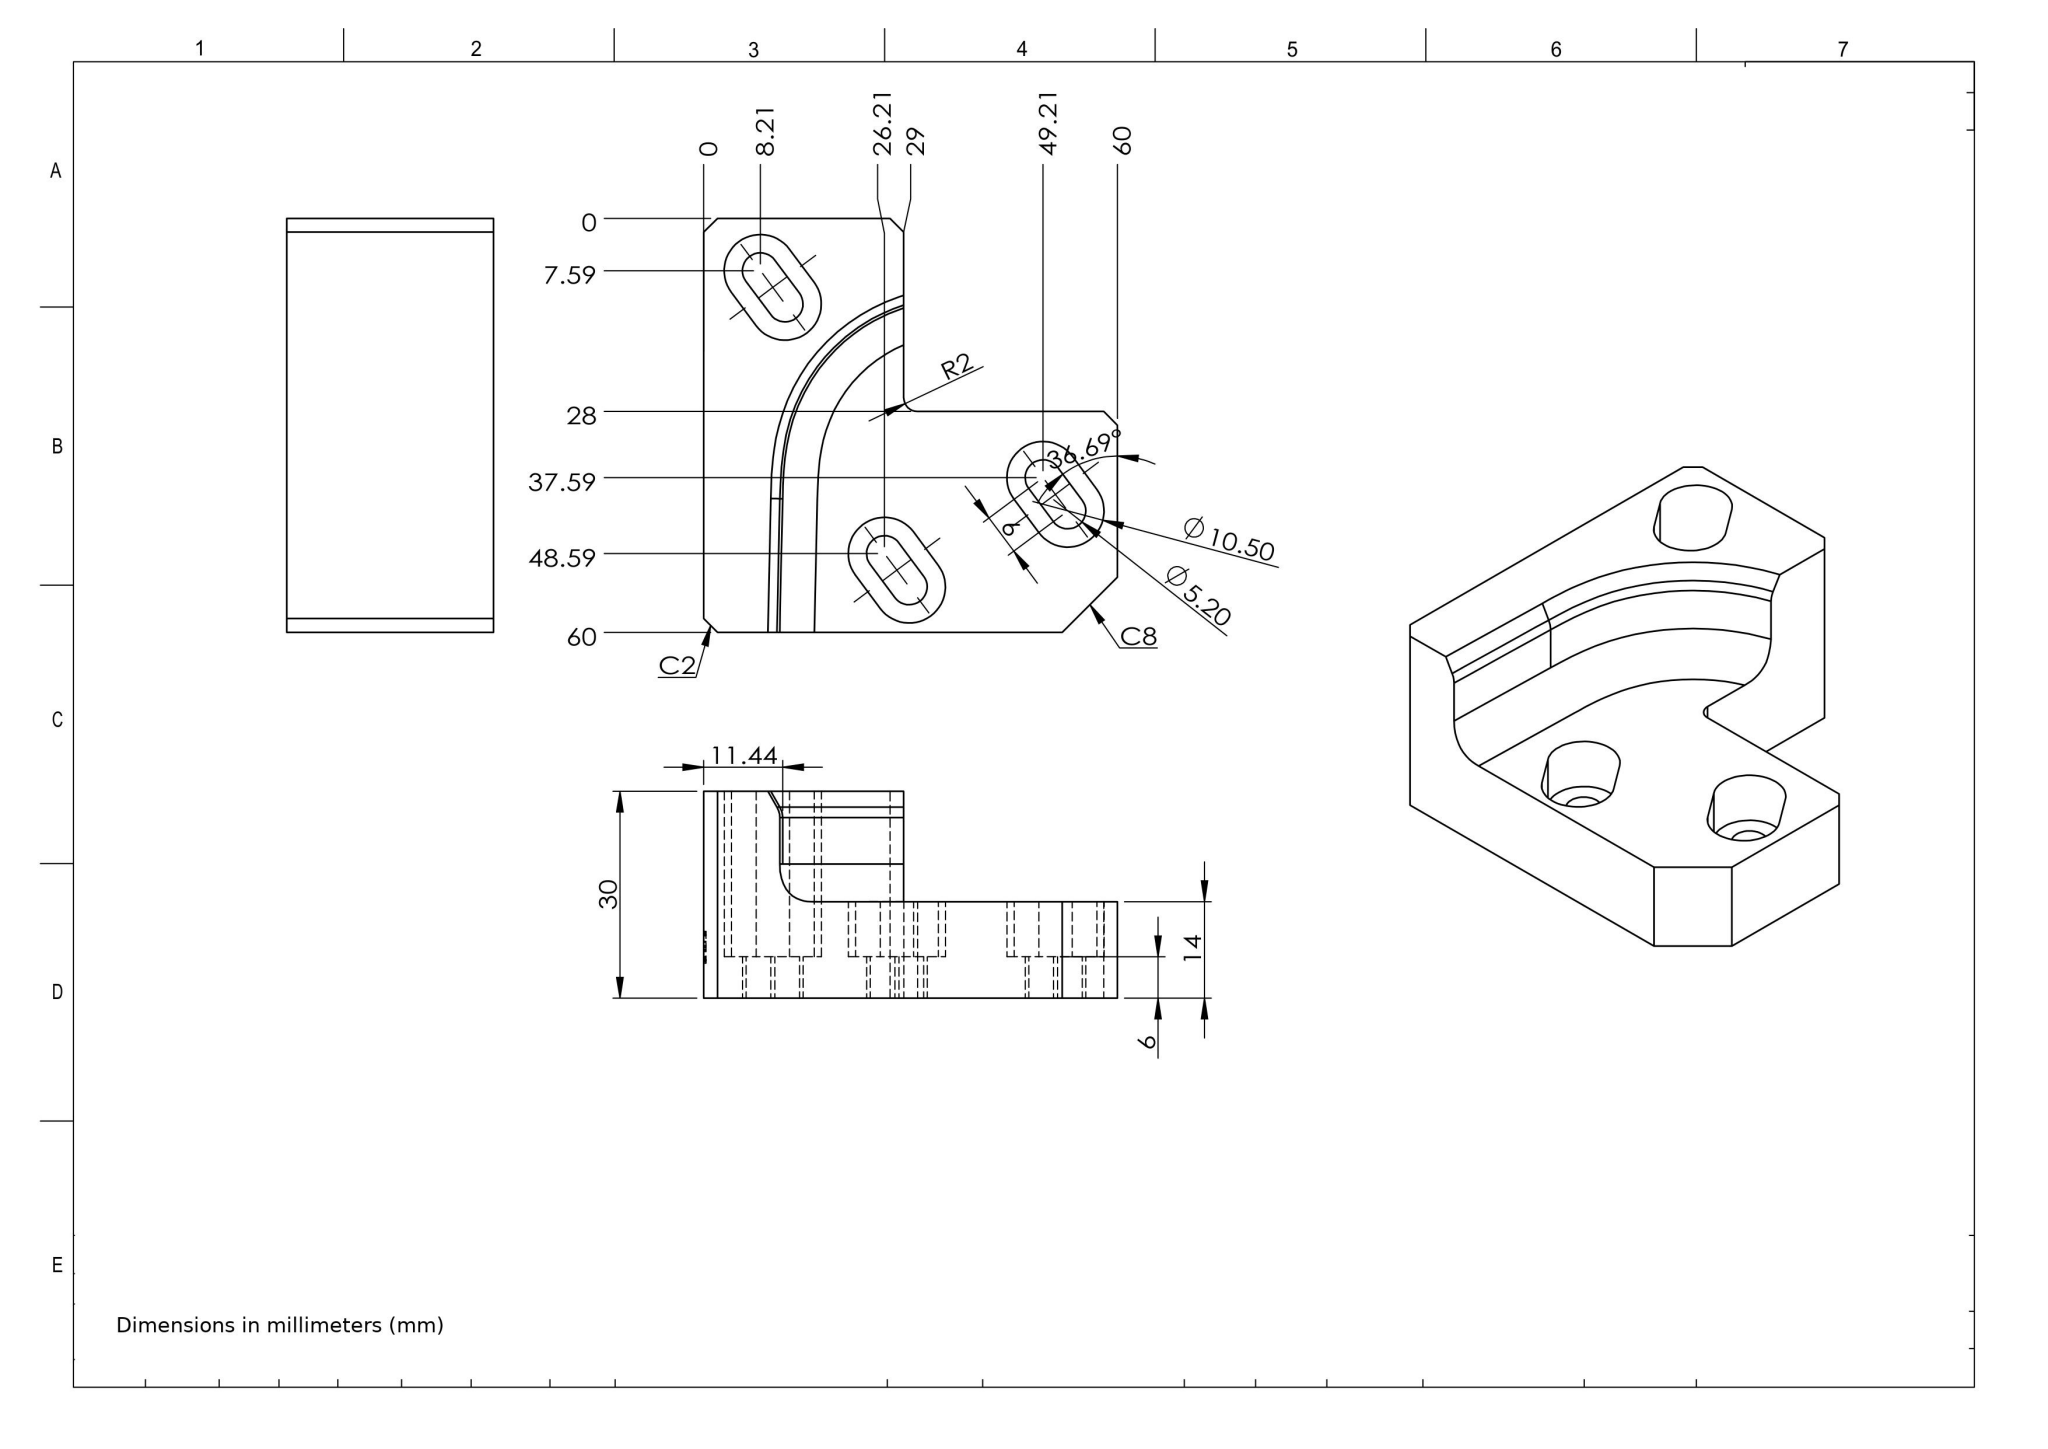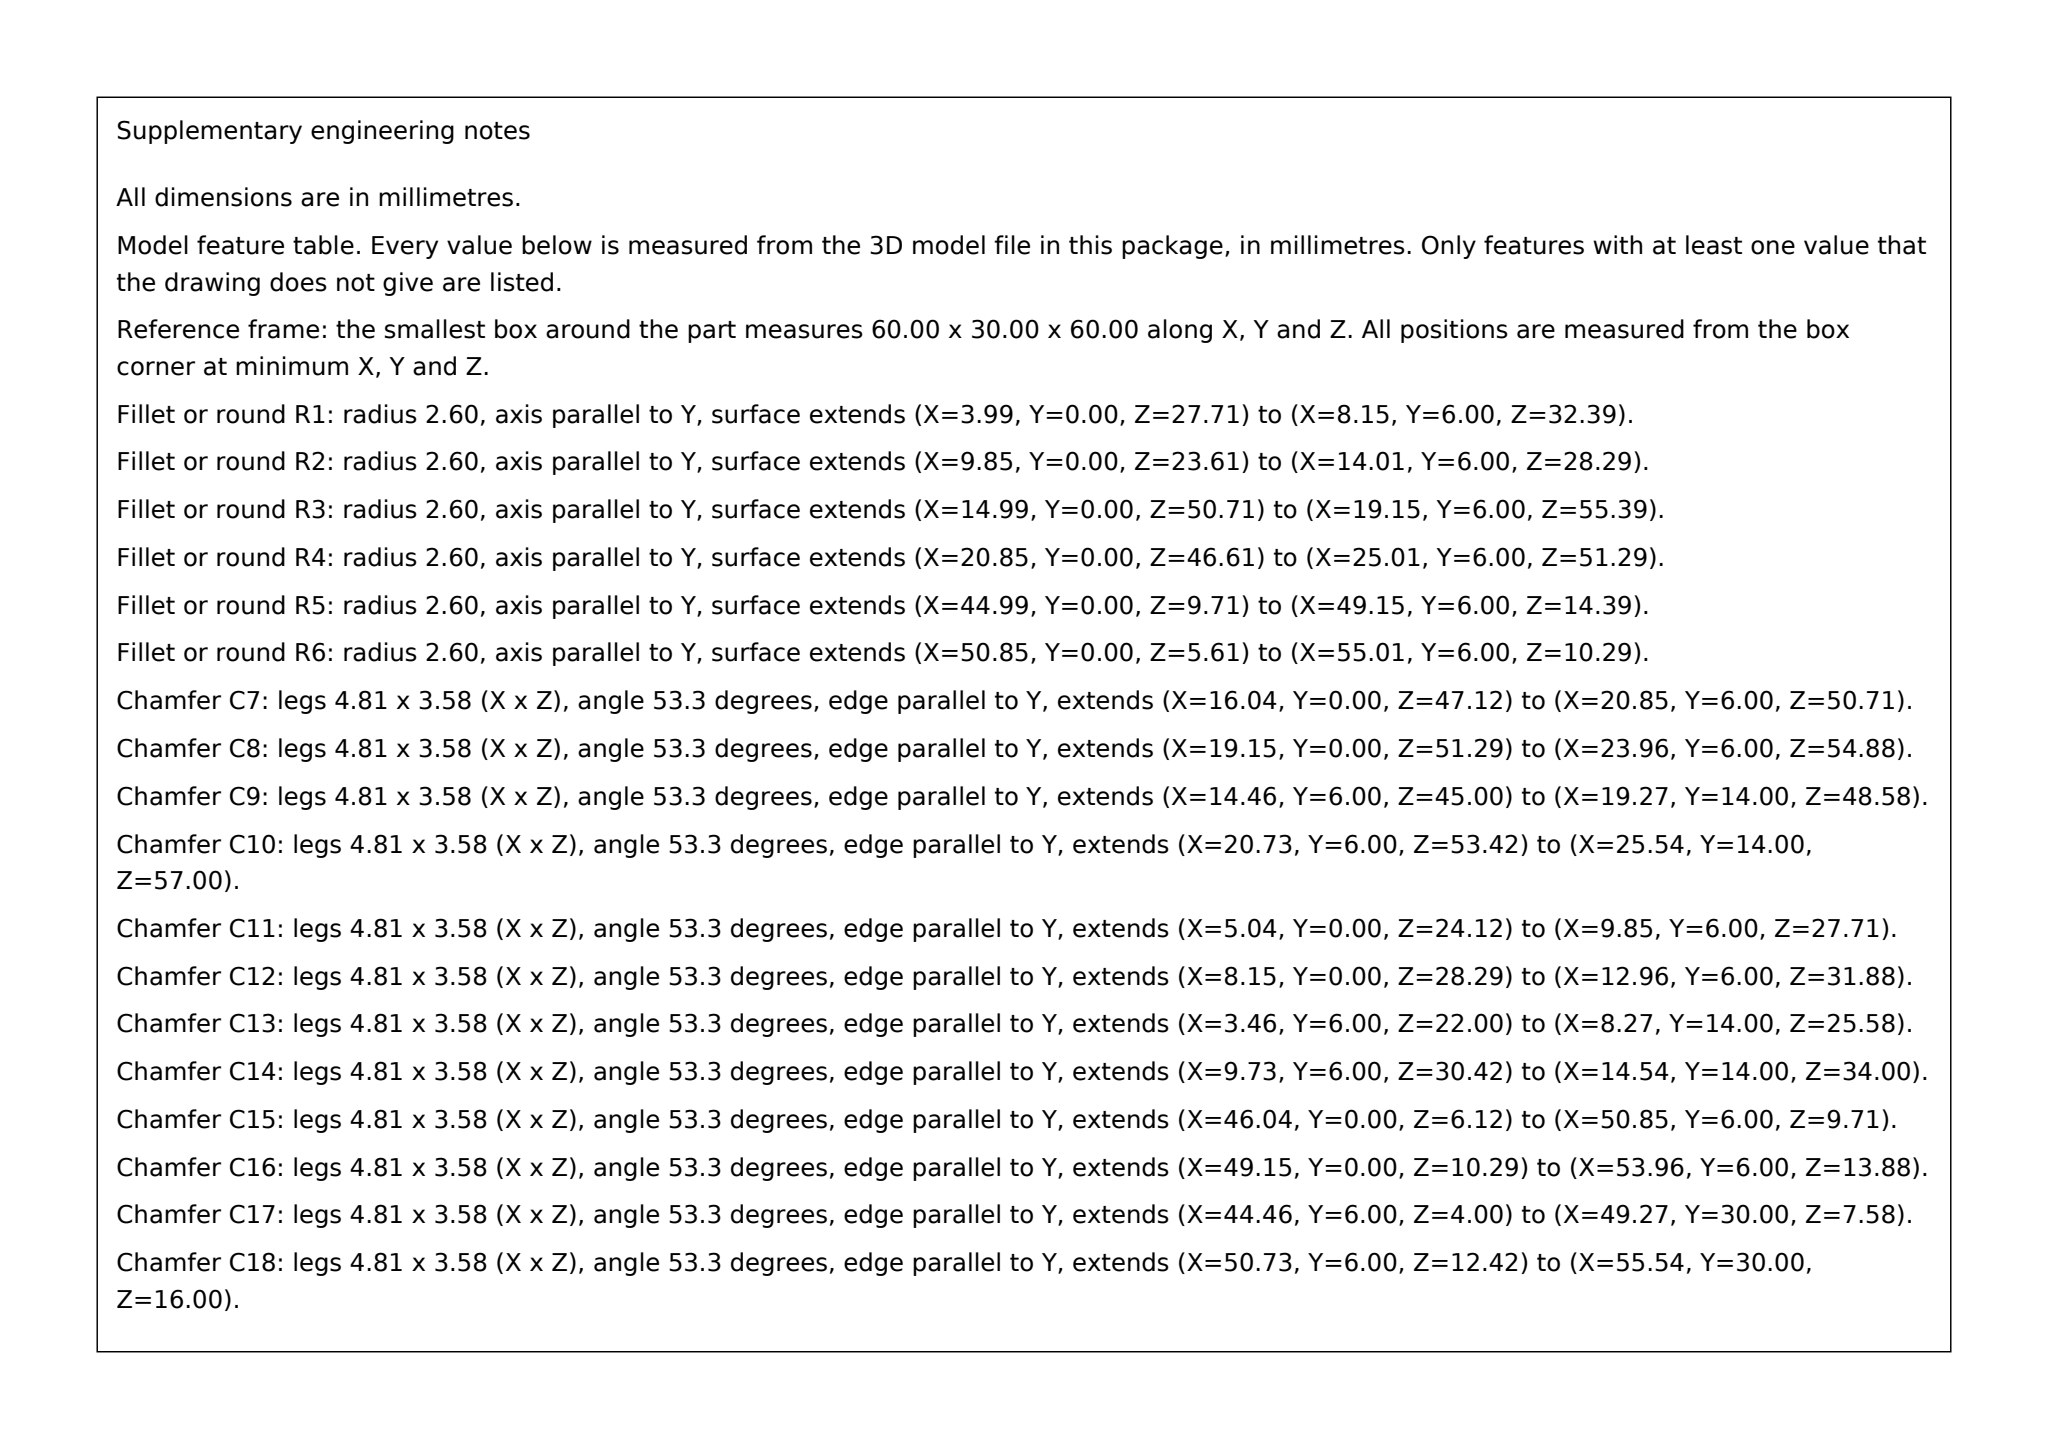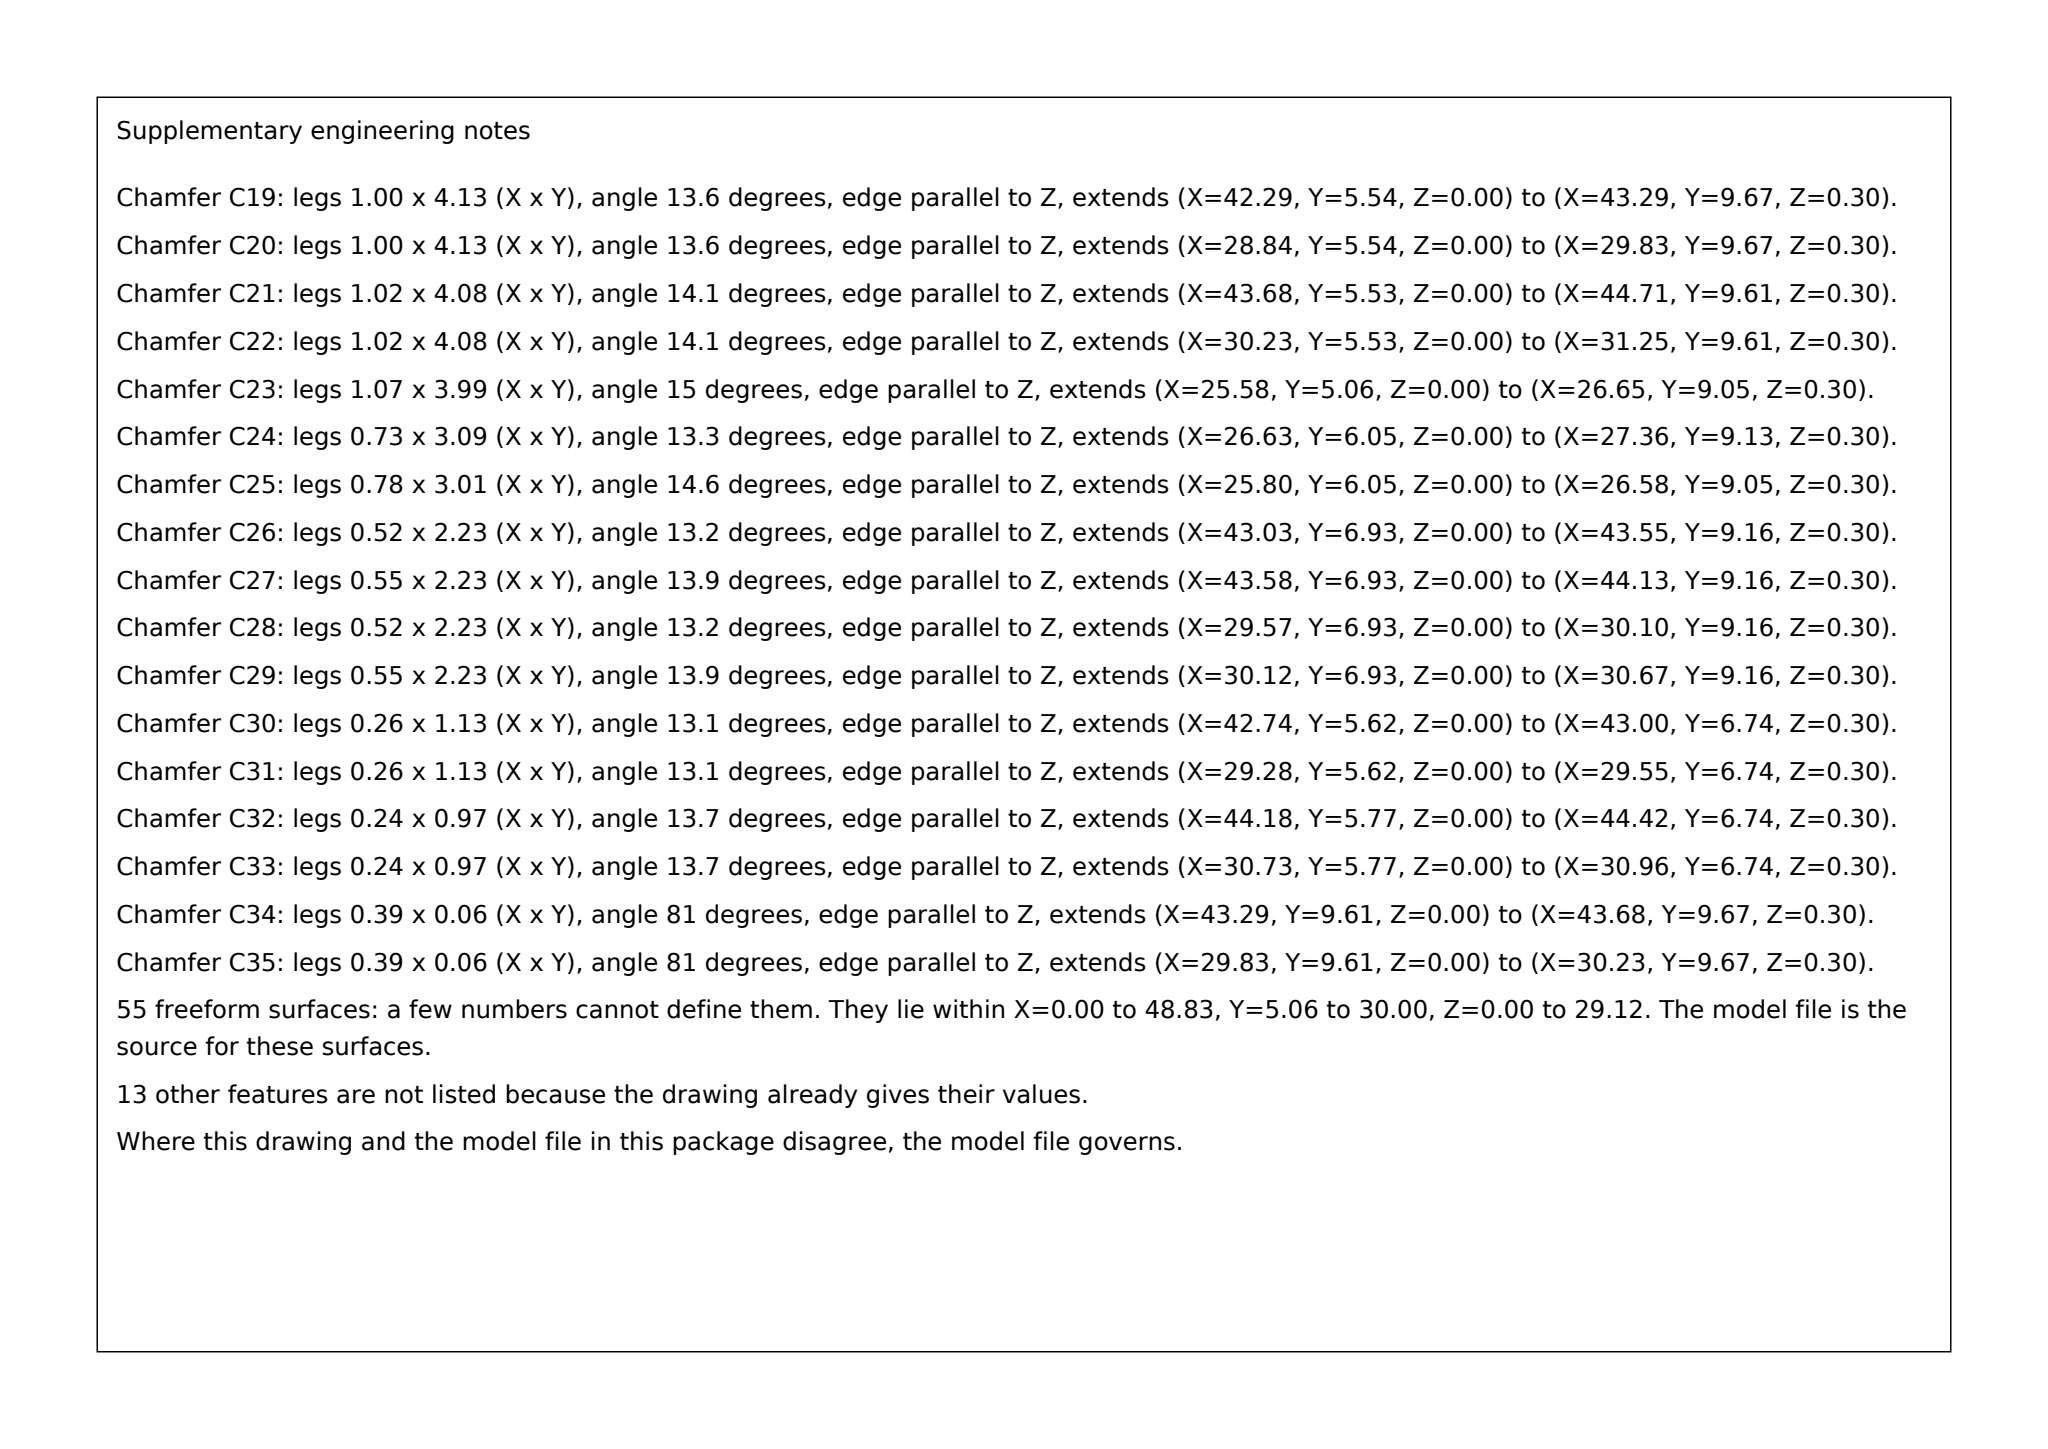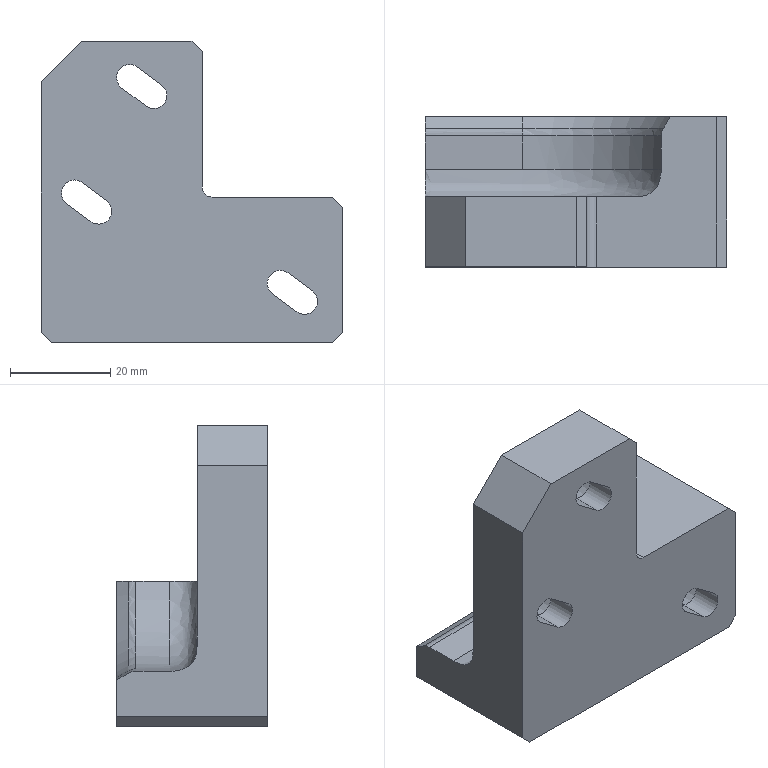Part | SolidWorks | mm | 1 solid | 226 faces | box 60 x 30 x 60 mm | volume 47215 mm3 | plane 152 | spline 55 | cylinder 19 | commonest cylinder face diameters 10.5 x9 5.2 x9 4 x1